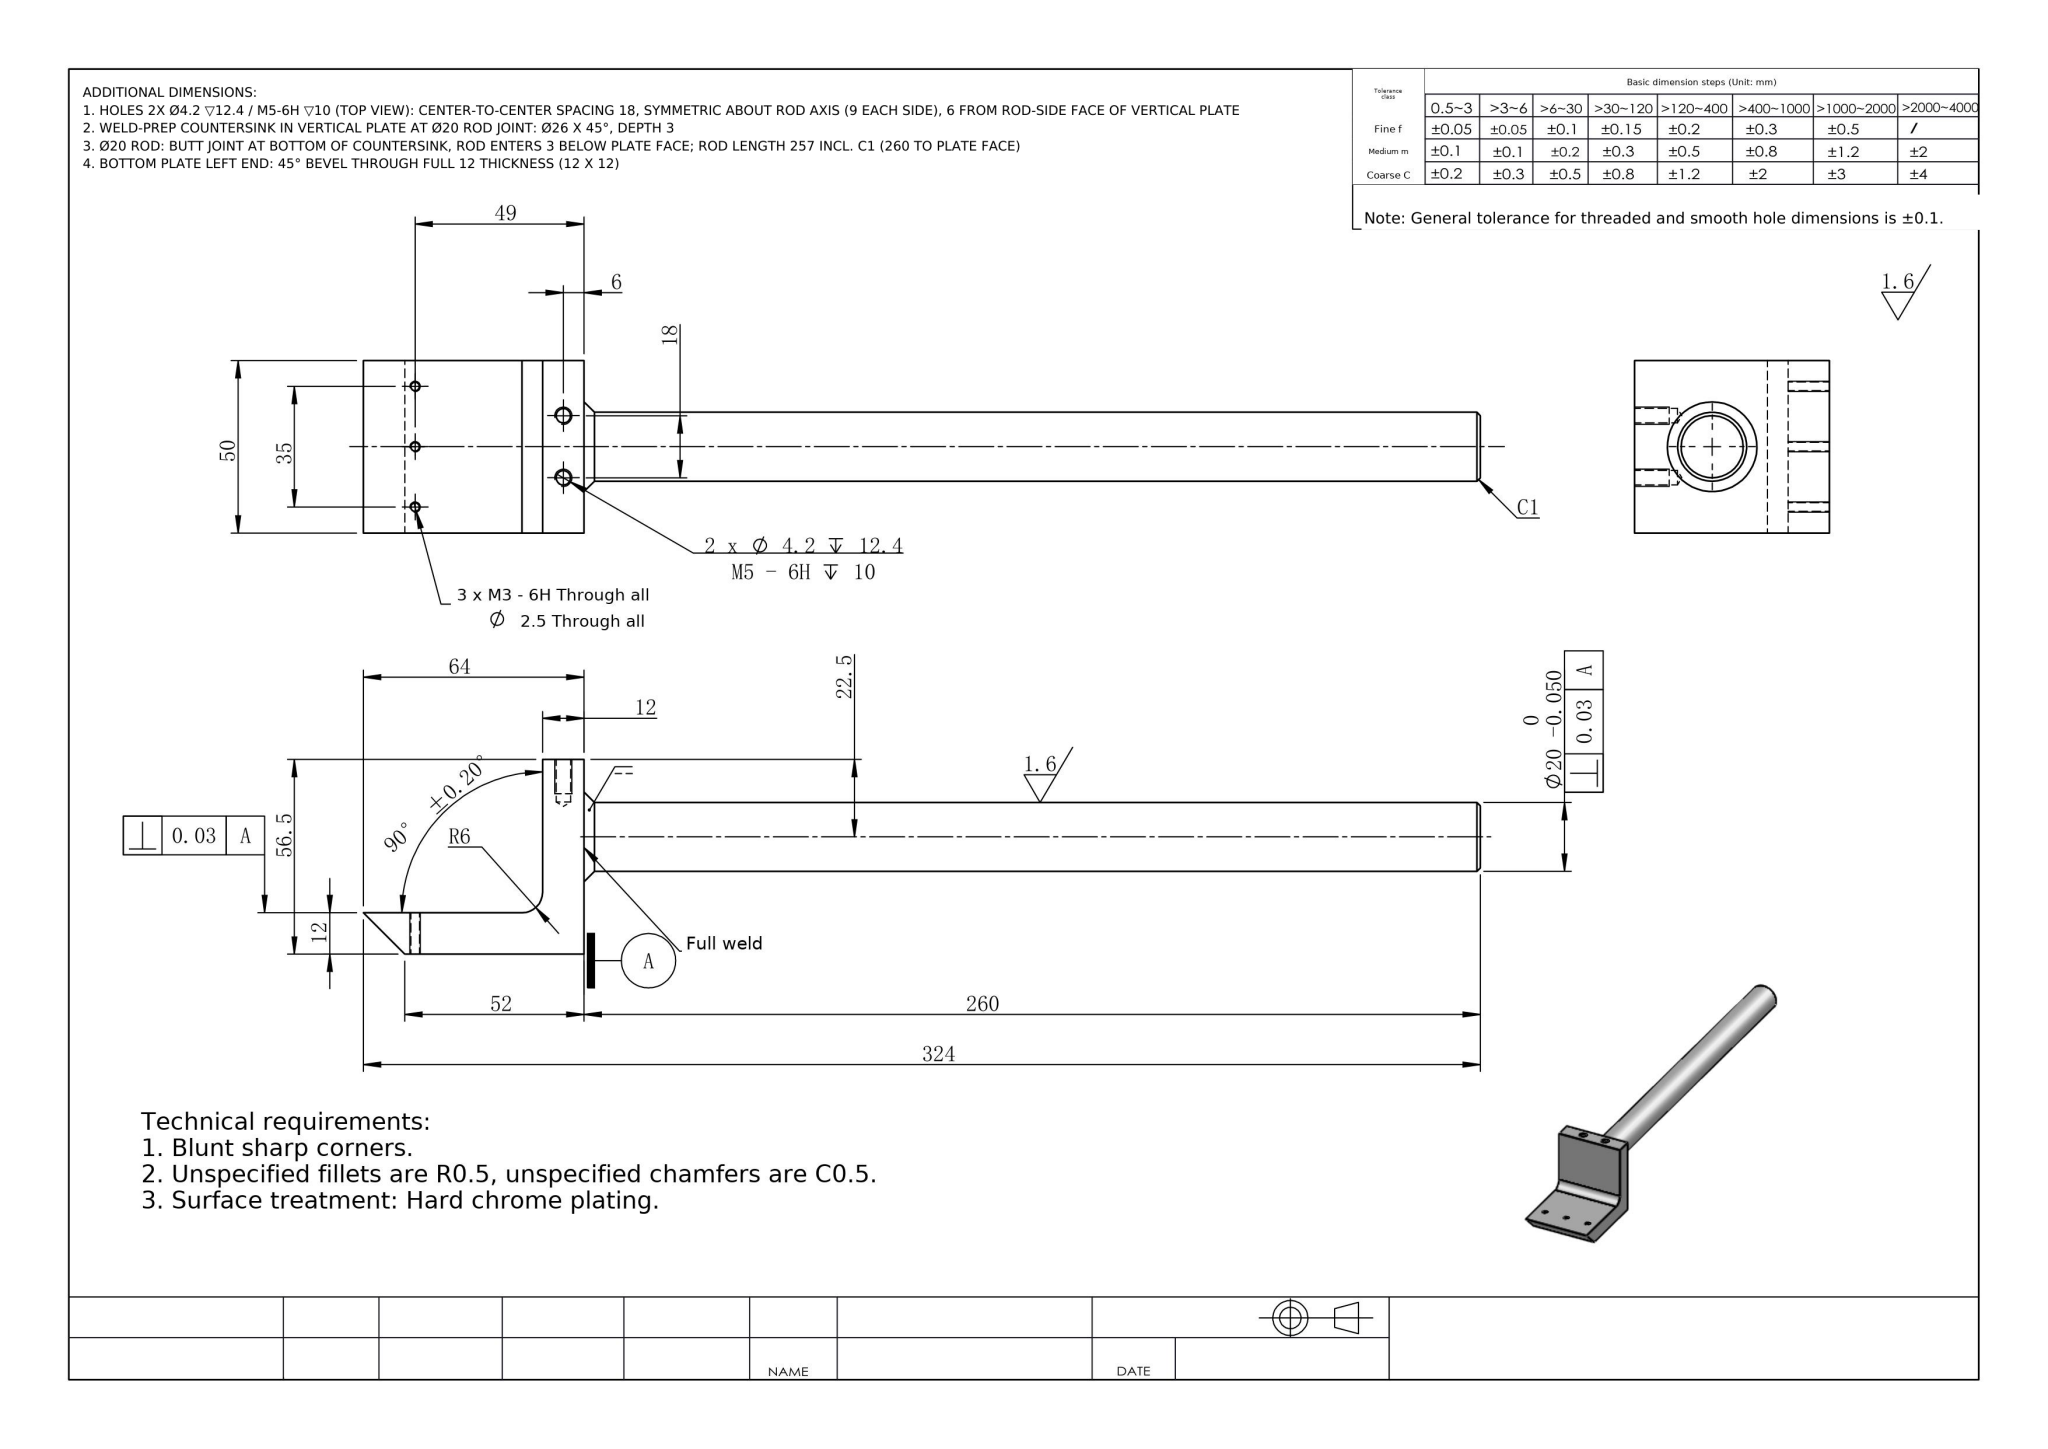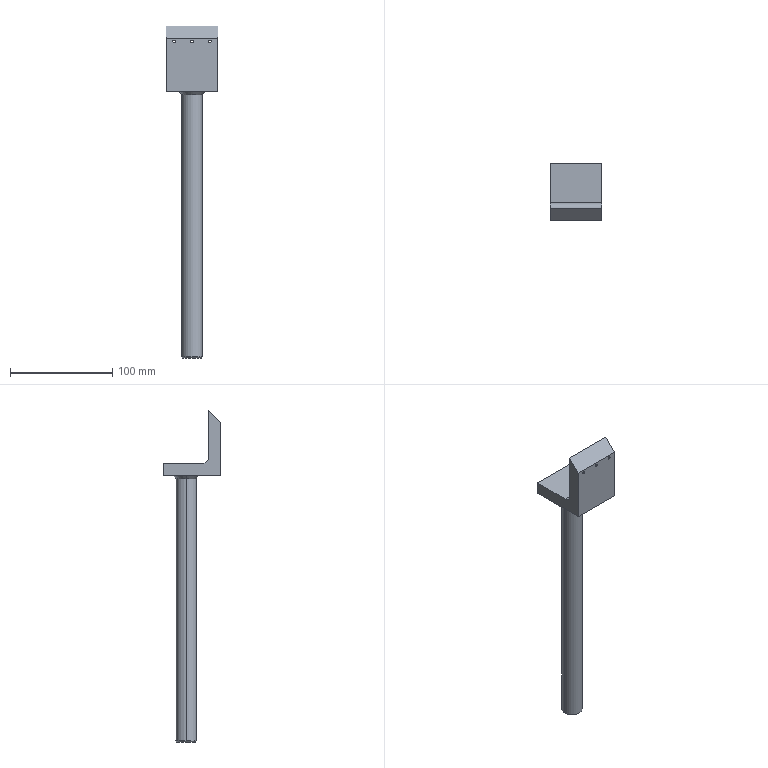Part | NX | mm | 1 solid | 30 faces | box 50 x 56.5 x 324 mm | volume 143316 mm3 | cylinder 13 | plane 9 | cone 8 | commonest cylinder face diameters 2.5 x6 4.2 x4 20 x2 12 x1